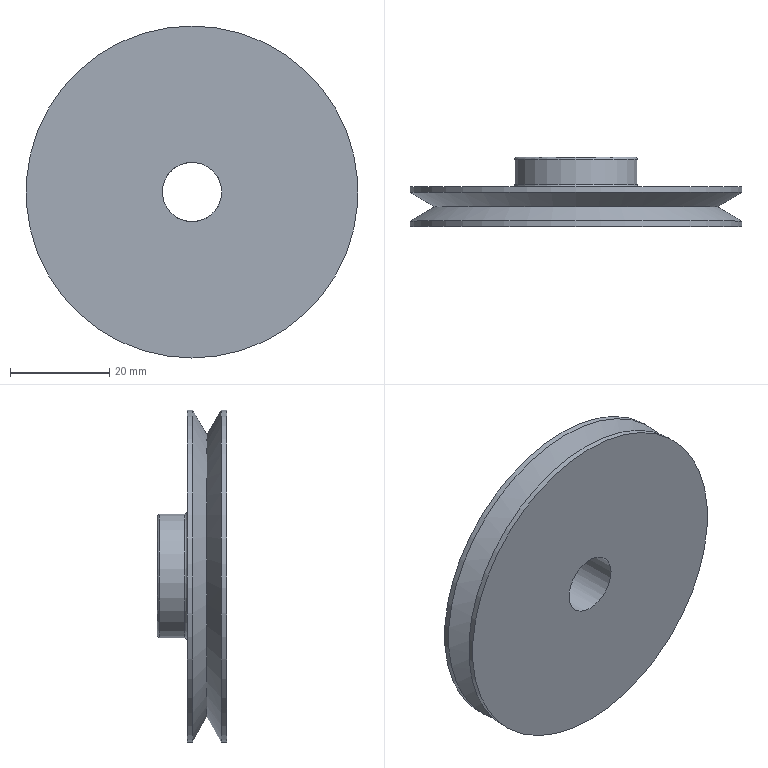Component | NX | PULLEY_2 | 1 solid | 11 faces | box 67 x 14 x 67 mm | volume 26680 mm3 | cylinder 4 | plane 3 | cone 2 | torus 2 | commonest cylinder face diameters 67 x2 25 x1 12 x1
STEP:
#1=CARTESIAN_POINT('',(0.,0.,0.));
#2=DIRECTION('',(0.,0.,1.));
#3=DIRECTION('',(1.,0.,0.));
#4=AXIS2_PLACEMENT_3D('',#1,#2,#3);
#5=CARTESIAN_POINT('',(-218.5,-55.,105.));
#6=VERTEX_POINT('',#5);
#7=CARTESIAN_POINT('',(-212.5,-55.,111.));
#8=VERTEX_POINT('',#7);
#9=CARTESIAN_POINT('',(-218.5,-55.,111.));
#10=DIRECTION('',(0.,-1.,0.));
#11=DIRECTION('',(0.,0.,-1.));
#12=AXIS2_PLACEMENT_3D('',#9,#10,#11);
#13=CIRCLE('',#12,6.);
#14=CARTESIAN_POINT('',(-218.5,-55.,144.5));
#15=DIRECTION('',(0.,-1.,0.));
#16=DIRECTION('',(0.,0.,-1.));
#17=AXIS2_PLACEMENT_3D('',#14,#15,#16);
#18=PLANE('',#17);
#19=CARTESIAN_POINT('',(33.5,0.));
#20=DIRECTION('',(1.,0.));
#21=AXIS2_PLACEMENT_2D('',#19,#20);
#22=CIRCLE('',#21,6.);
#23=(GEOMETRIC_REPRESENTATION_CONTEXT(2)PARAMETRIC_REPRESENTATION_CONTEXT()REPRESENTATION_CONTEXT('',''));
#24=DEFINITIONAL_REPRESENTATION('',(#22),#23);
#25=PCURVE('',#18,#24);
#26=CARTESIAN_POINT('',(-218.5,-96.,111.));
#27=DIRECTION('',(0.,1.,0.));
#28=DIRECTION('',(0.,0.,1.));
#29=AXIS2_PLACEMENT_3D('',#26,#27,#28);
#30=CYLINDRICAL_SURFACE('',#29,6.);
#31=CARTESIAN_POINT('',(3.142,41.));
#32=DIRECTION('',(-1.,0.));
#33=VECTOR('',#32,1.);
#34=LINE('',#31,#33);
#35=(GEOMETRIC_REPRESENTATION_CONTEXT(2)PARAMETRIC_REPRESENTATION_CONTEXT()REPRESENTATION_CONTEXT('',''));
#36=DEFINITIONAL_REPRESENTATION('',(#34),#35);
#37=PCURVE('',#30,#36);
#38=SURFACE_CURVE('',#13,(#25,#37),.PCURVE_S1.);
#39=EDGE_CURVE('',#6,#8,#38,.T.);
#40=ORIENTED_EDGE('',*,*,#39,.F.);
#41=CARTESIAN_POINT('',(-218.5,-55.,111.));
#42=DIRECTION('',(0.,-1.,0.));
#43=DIRECTION('',(0.,0.,-1.));
#44=AXIS2_PLACEMENT_3D('',#41,#42,#43);
#45=CIRCLE('',#44,6.);
#46=CARTESIAN_POINT('',(33.5,0.));
#47=DIRECTION('',(1.,0.));
#48=AXIS2_PLACEMENT_2D('',#46,#47);
#49=CIRCLE('',#48,6.);
#50=(GEOMETRIC_REPRESENTATION_CONTEXT(2)PARAMETRIC_REPRESENTATION_CONTEXT()REPRESENTATION_CONTEXT('',''));
#51=DEFINITIONAL_REPRESENTATION('',(#49),#50);
#52=PCURVE('',#18,#51);
#53=CARTESIAN_POINT('',(9.425,41.));
#54=DIRECTION('',(-1.,0.));
#55=VECTOR('',#54,1.);
#56=LINE('',#53,#55);
#57=(GEOMETRIC_REPRESENTATION_CONTEXT(2)PARAMETRIC_REPRESENTATION_CONTEXT()REPRESENTATION_CONTEXT('',''));
#58=DEFINITIONAL_REPRESENTATION('',(#56),#57);
#59=PCURVE('',#30,#58);
#60=SURFACE_CURVE('',#45,(#52,#59),.PCURVE_S1.);
#61=EDGE_CURVE('',#8,#6,#60,.T.);
#62=ORIENTED_EDGE('',*,*,#61,.F.);
#63=EDGE_LOOP('',(#40,#62));
#64=FACE_BOUND('',#63,.T.);
#65=CARTESIAN_POINT('',(-218.5,-55.,144.5));
#66=VERTEX_POINT('',#65);
#67=CARTESIAN_POINT('',(-218.5,-55.,111.));
#68=DIRECTION('',(0.,1.,0.));
#69=DIRECTION('',(0.,0.,1.));
#70=AXIS2_PLACEMENT_3D('',#67,#68,#69);
#71=CIRCLE('',#70,33.5);
#72=CARTESIAN_POINT('',(0.,0.));
#73=CARTESIAN_POINT('',(0.,58.024));
#74=CARTESIAN_POINT('',(50.25,29.012));
#75=CARTESIAN_POINT('',(100.5,0.));
#76=CARTESIAN_POINT('',(50.25,-29.012));
#77=CARTESIAN_POINT('',(0.,-58.024));
#78=CARTESIAN_POINT('',(0.,0.));
#79=(BOUNDED_CURVE()B_SPLINE_CURVE(2,(#72,#73,#74,#75,#76,#77,#78),.UNSPECIFIED.,.T.,.F.)B_SPLINE_CURVE_WITH_KNOTS((1,2,2,2,2,1),(-2.094,0.,2.094,4.189,6.283,8.378),.UNSPECIFIED.)CURVE()GEOMETRIC_REPRESENTATION_ITEM()RATIONAL_B_SPLINE_CURVE((1.,0.5,1.,0.5,1.,0.5,1.))REPRESENTATION_ITEM(''));
#80=(GEOMETRIC_REPRESENTATION_CONTEXT(2)PARAMETRIC_REPRESENTATION_CONTEXT()REPRESENTATION_CONTEXT('',''));
#81=DEFINITIONAL_REPRESENTATION('',(#79),#80);
#82=PCURVE('',#18,#81);
#83=CARTESIAN_POINT('',(-218.5,-51.,111.));
#84=DIRECTION('',(0.,1.,0.));
#85=DIRECTION('',(0.,0.,1.));
#86=AXIS2_PLACEMENT_3D('',#83,#84,#85);
#87=CYLINDRICAL_SURFACE('',#86,33.5);
#88=CARTESIAN_POINT('',(0.,-4.));
#89=DIRECTION('',(1.,0.));
#90=VECTOR('',#89,1.);
#91=LINE('',#88,#90);
#92=(GEOMETRIC_REPRESENTATION_CONTEXT(2)PARAMETRIC_REPRESENTATION_CONTEXT()REPRESENTATION_CONTEXT('',''));
#93=DEFINITIONAL_REPRESENTATION('',(#91),#92);
#94=PCURVE('',#87,#93);
#95=SURFACE_CURVE('',#71,(#82,#94),.PCURVE_S1.);
#96=EDGE_CURVE('',#66,#66,#95,.T.);
#97=ORIENTED_EDGE('',*,*,#96,.F.);
#98=EDGE_LOOP('',(#97));
#99=FACE_BOUND('',#98,.T.);
#100=ADVANCED_FACE('',(#64,#99),#18,.T.);
#101=ORIENTED_EDGE('',*,*,#96,.T.);
#102=CARTESIAN_POINT('',(-218.5,-53.887,144.5));
#103=VERTEX_POINT('',#102);
#104=CARTESIAN_POINT('',(-218.5,-55.,144.5));
#105=CARTESIAN_POINT('',(-218.5,-53.887,144.5));
#106=B_SPLINE_CURVE_WITH_KNOTS('',1,(#104,#105),.UNSPECIFIED.,.F.,.F.,(2,2),(-4.,-2.887),.PIECEWISE_BEZIER_KNOTS.);
#107=CARTESIAN_POINT('',(6.283,0.));
#108=DIRECTION('',(0.,1.));
#109=VECTOR('',#108,1.);
#110=LINE('',#107,#109);
#111=(GEOMETRIC_REPRESENTATION_CONTEXT(2)PARAMETRIC_REPRESENTATION_CONTEXT()REPRESENTATION_CONTEXT('',''));
#112=DEFINITIONAL_REPRESENTATION('',(#110),#111);
#113=PCURVE('',#87,#112);
#114=CARTESIAN_POINT('',(0.,0.));
#115=DIRECTION('',(0.,1.));
#116=VECTOR('',#115,1.);
#117=LINE('',#114,#116);
#118=(GEOMETRIC_REPRESENTATION_CONTEXT(2)PARAMETRIC_REPRESENTATION_CONTEXT()REPRESENTATION_CONTEXT('',''));
#119=DEFINITIONAL_REPRESENTATION('',(#117),#118);
#120=PCURVE('',#87,#119);
#121=SEAM_CURVE('',#106,(#113,#120),.PCURVE_S1.);
#122=EDGE_CURVE('',#66,#103,#121,.T.);
#123=ORIENTED_EDGE('',*,*,#122,.T.);
#124=CARTESIAN_POINT('',(-218.5,-53.887,111.));
#125=DIRECTION('',(0.,1.,0.));
#126=DIRECTION('',(0.,0.,1.));
#127=AXIS2_PLACEMENT_3D('',#124,#125,#126);
#128=CIRCLE('',#127,33.5);
#129=CARTESIAN_POINT('',(0.,-2.887));
#130=DIRECTION('',(1.,0.));
#131=VECTOR('',#130,1.);
#132=LINE('',#129,#131);
#133=(GEOMETRIC_REPRESENTATION_CONTEXT(2)PARAMETRIC_REPRESENTATION_CONTEXT()REPRESENTATION_CONTEXT('',''));
#134=DEFINITIONAL_REPRESENTATION('',(#132),#133);
#135=PCURVE('',#87,#134);
#136=CARTESIAN_POINT('',(-218.5,-51.,111.));
#137=DIRECTION('',(0.,-1.,0.));
#138=DIRECTION('',(0.,0.,-1.));
#139=AXIS2_PLACEMENT_3D('',#136,#137,#138);
#140=CONICAL_SURFACE('',#139,28.5,1.047);
#141=CARTESIAN_POINT('',(9.425,2.887));
#142=DIRECTION('',(-1.,0.));
#143=VECTOR('',#142,1.);
#144=LINE('',#141,#143);
#145=(GEOMETRIC_REPRESENTATION_CONTEXT(2)PARAMETRIC_REPRESENTATION_CONTEXT()REPRESENTATION_CONTEXT('',''));
#146=DEFINITIONAL_REPRESENTATION('',(#144),#145);
#147=PCURVE('',#140,#146);
#148=SURFACE_CURVE('',#128,(#135,#147),.PCURVE_S1.);
#149=EDGE_CURVE('',#103,#103,#148,.T.);
#150=ORIENTED_EDGE('',*,*,#149,.F.);
#151=ORIENTED_EDGE('',*,*,#122,.F.);
#152=EDGE_LOOP('',(#101,#123,#150,#151));
#153=FACE_BOUND('',#152,.T.);
#154=ADVANCED_FACE('',(#153),#87,.T.);
#155=ORIENTED_EDGE('',*,*,#149,.T.);
#156=CARTESIAN_POINT('',(-218.5,-51.,139.5));
#157=VERTEX_POINT('',#156);
#158=CARTESIAN_POINT('',(-218.5,-51.,139.5));
#159=CARTESIAN_POINT('',(-218.5,-53.887,144.5));
#160=B_SPLINE_CURVE_WITH_KNOTS('',1,(#158,#159),.UNSPECIFIED.,.F.,.F.,(2,2),(0.,5.774),.PIECEWISE_BEZIER_KNOTS.);
#161=CARTESIAN_POINT('',(3.142,0.));
#162=DIRECTION('',(0.,1.));
#163=VECTOR('',#162,1.);
#164=LINE('',#161,#163);
#165=(GEOMETRIC_REPRESENTATION_CONTEXT(2)PARAMETRIC_REPRESENTATION_CONTEXT()REPRESENTATION_CONTEXT('',''));
#166=DEFINITIONAL_REPRESENTATION('',(#164),#165);
#167=PCURVE('',#140,#166);
#168=CARTESIAN_POINT('',(9.425,0.));
#169=DIRECTION('',(0.,1.));
#170=VECTOR('',#169,1.);
#171=LINE('',#168,#170);
#172=(GEOMETRIC_REPRESENTATION_CONTEXT(2)PARAMETRIC_REPRESENTATION_CONTEXT()REPRESENTATION_CONTEXT('',''));
#173=DEFINITIONAL_REPRESENTATION('',(#171),#172);
#174=PCURVE('',#140,#173);
#175=SEAM_CURVE('',#160,(#167,#174),.PCURVE_S1.);
#176=EDGE_CURVE('',#157,#103,#175,.T.);
#177=ORIENTED_EDGE('',*,*,#176,.F.);
#178=CARTESIAN_POINT('',(-218.5,-51.,111.));
#179=DIRECTION('',(0.,1.,0.));
#180=DIRECTION('',(0.,0.,1.));
#181=AXIS2_PLACEMENT_3D('',#178,#179,#180);
#182=CIRCLE('',#181,28.5);
#183=CARTESIAN_POINT('',(9.425,0.));
#184=DIRECTION('',(-1.,0.));
#185=VECTOR('',#184,1.);
#186=LINE('',#183,#185);
#187=(GEOMETRIC_REPRESENTATION_CONTEXT(2)PARAMETRIC_REPRESENTATION_CONTEXT()REPRESENTATION_CONTEXT('',''));
#188=DEFINITIONAL_REPRESENTATION('',(#186),#187);
#189=PCURVE('',#140,#188);
#190=CARTESIAN_POINT('',(-218.5,-48.113,111.));
#191=DIRECTION('',(0.,1.,0.));
#192=DIRECTION('',(0.,0.,1.));
#193=AXIS2_PLACEMENT_3D('',#190,#191,#192);
#194=CONICAL_SURFACE('',#193,33.5,1.047);
#195=CARTESIAN_POINT('',(0.,-2.887));
#196=DIRECTION('',(1.,0.));
#197=VECTOR('',#196,1.);
#198=LINE('',#195,#197);
#199=(GEOMETRIC_REPRESENTATION_CONTEXT(2)PARAMETRIC_REPRESENTATION_CONTEXT()REPRESENTATION_CONTEXT('',''));
#200=DEFINITIONAL_REPRESENTATION('',(#198),#199);
#201=PCURVE('',#194,#200);
#202=SURFACE_CURVE('',#182,(#189,#201),.PCURVE_S1.);
#203=EDGE_CURVE('',#157,#157,#202,.T.);
#204=ORIENTED_EDGE('',*,*,#203,.F.);
#205=ORIENTED_EDGE('',*,*,#176,.T.);
#206=EDGE_LOOP('',(#155,#177,#204,#205));
#207=FACE_BOUND('',#206,.T.);
#208=ADVANCED_FACE('',(#207),#140,.T.);
#209=ORIENTED_EDGE('',*,*,#203,.T.);
#210=CARTESIAN_POINT('',(-218.5,-48.113,144.5));
#211=VERTEX_POINT('',#210);
#212=CARTESIAN_POINT('',(-218.5,-51.,139.5));
#213=CARTESIAN_POINT('',(-218.5,-48.113,144.5));
#214=B_SPLINE_CURVE_WITH_KNOTS('',1,(#212,#213),.UNSPECIFIED.,.F.,.F.,(2,2),(-5.774,0.),.PIECEWISE_BEZIER_KNOTS.);
#215=CARTESIAN_POINT('',(6.283,0.));
#216=DIRECTION('',(0.,1.));
#217=VECTOR('',#216,1.);
#218=LINE('',#215,#217);
#219=(GEOMETRIC_REPRESENTATION_CONTEXT(2)PARAMETRIC_REPRESENTATION_CONTEXT()REPRESENTATION_CONTEXT('',''));
#220=DEFINITIONAL_REPRESENTATION('',(#218),#219);
#221=PCURVE('',#194,#220);
#222=CARTESIAN_POINT('',(0.,0.));
#223=DIRECTION('',(0.,1.));
#224=VECTOR('',#223,1.);
#225=LINE('',#222,#224);
#226=(GEOMETRIC_REPRESENTATION_CONTEXT(2)PARAMETRIC_REPRESENTATION_CONTEXT()REPRESENTATION_CONTEXT('',''));
#227=DEFINITIONAL_REPRESENTATION('',(#225),#226);
#228=PCURVE('',#194,#227);
#229=SEAM_CURVE('',#214,(#221,#228),.PCURVE_S1.);
#230=EDGE_CURVE('',#157,#211,#229,.T.);
#231=ORIENTED_EDGE('',*,*,#230,.T.);
#232=CARTESIAN_POINT('',(-218.5,-48.113,111.));
#233=DIRECTION('',(0.,1.,0.));
#234=DIRECTION('',(0.,0.,1.));
#235=AXIS2_PLACEMENT_3D('',#232,#233,#234);
#236=CIRCLE('',#235,33.5);
#237=CARTESIAN_POINT('',(0.,0.));
#238=DIRECTION('',(1.,0.));
#239=VECTOR('',#238,1.);
#240=LINE('',#237,#239);
#241=(GEOMETRIC_REPRESENTATION_CONTEXT(2)PARAMETRIC_REPRESENTATION_CONTEXT()REPRESENTATION_CONTEXT('',''));
#242=DEFINITIONAL_REPRESENTATION('',(#240),#241);
#243=PCURVE('',#194,#242);
#244=CARTESIAN_POINT('',(-218.5,-51.,111.));
#245=DIRECTION('',(0.,1.,0.));
#246=DIRECTION('',(0.,0.,1.));
#247=AXIS2_PLACEMENT_3D('',#244,#245,#246);
#248=CYLINDRICAL_SURFACE('',#247,33.5);
#249=CARTESIAN_POINT('',(0.,2.887));
#250=DIRECTION('',(1.,0.));
#251=VECTOR('',#250,1.);
#252=LINE('',#249,#251);
#253=(GEOMETRIC_REPRESENTATION_CONTEXT(2)PARAMETRIC_REPRESENTATION_CONTEXT()REPRESENTATION_CONTEXT('',''));
#254=DEFINITIONAL_REPRESENTATION('',(#252),#253);
#255=PCURVE('',#248,#254);
#256=SURFACE_CURVE('',#236,(#243,#255),.PCURVE_S1.);
#257=EDGE_CURVE('',#211,#211,#256,.T.);
#258=ORIENTED_EDGE('',*,*,#257,.F.);
#259=ORIENTED_EDGE('',*,*,#230,.F.);
#260=EDGE_LOOP('',(#209,#231,#258,#259));
#261=FACE_BOUND('',#260,.T.);
#262=ADVANCED_FACE('',(#261),#194,.T.);
#263=ORIENTED_EDGE('',*,*,#257,.T.);
#264=CARTESIAN_POINT('',(-218.5,-47.,144.5));
#265=VERTEX_POINT('',#264);
#266=CARTESIAN_POINT('',(-218.5,-48.113,144.5));
#267=CARTESIAN_POINT('',(-218.5,-47.,144.5));
#268=B_SPLINE_CURVE_WITH_KNOTS('',1,(#266,#267),.UNSPECIFIED.,.F.,.F.,(2,2),(2.887,4.),.PIECEWISE_BEZIER_KNOTS.);
#269=CARTESIAN_POINT('',(6.283,0.));
#270=DIRECTION('',(0.,1.));
#271=VECTOR('',#270,1.);
#272=LINE('',#269,#271);
#273=(GEOMETRIC_REPRESENTATION_CONTEXT(2)PARAMETRIC_REPRESENTATION_CONTEXT()REPRESENTATION_CONTEXT('',''));
#274=DEFINITIONAL_REPRESENTATION('',(#272),#273);
#275=PCURVE('',#248,#274);
#276=CARTESIAN_POINT('',(0.,0.));
#277=DIRECTION('',(0.,1.));
#278=VECTOR('',#277,1.);
#279=LINE('',#276,#278);
#280=(GEOMETRIC_REPRESENTATION_CONTEXT(2)PARAMETRIC_REPRESENTATION_CONTEXT()REPRESENTATION_CONTEXT('',''));
#281=DEFINITIONAL_REPRESENTATION('',(#279),#280);
#282=PCURVE('',#248,#281);
#283=SEAM_CURVE('',#268,(#275,#282),.PCURVE_S1.);
#284=EDGE_CURVE('',#211,#265,#283,.T.);
#285=ORIENTED_EDGE('',*,*,#284,.T.);
#286=CARTESIAN_POINT('',(-218.5,-47.,111.));
#287=DIRECTION('',(0.,1.,0.));
#288=DIRECTION('',(0.,0.,1.));
#289=AXIS2_PLACEMENT_3D('',#286,#287,#288);
#290=CIRCLE('',#289,33.5);
#291=CARTESIAN_POINT('',(0.,4.));
#292=DIRECTION('',(1.,0.));
#293=VECTOR('',#292,1.);
#294=LINE('',#291,#293);
#295=(GEOMETRIC_REPRESENTATION_CONTEXT(2)PARAMETRIC_REPRESENTATION_CONTEXT()REPRESENTATION_CONTEXT('',''));
#296=DEFINITIONAL_REPRESENTATION('',(#294),#295);
#297=PCURVE('',#248,#296);
#298=CARTESIAN_POINT('',(-218.5,-47.,111.));
#299=DIRECTION('',(0.,1.,0.));
#300=DIRECTION('',(0.,0.,1.));
#301=AXIS2_PLACEMENT_3D('',#298,#299,#300);
#302=PLANE('',#301);
#303=CARTESIAN_POINT('',(0.,0.));
#304=DIRECTION('',(1.,0.));
#305=AXIS2_PLACEMENT_2D('',#303,#304);
#306=CIRCLE('',#305,33.5);
#307=(GEOMETRIC_REPRESENTATION_CONTEXT(2)PARAMETRIC_REPRESENTATION_CONTEXT()REPRESENTATION_CONTEXT('',''));
#308=DEFINITIONAL_REPRESENTATION('',(#306),#307);
#309=PCURVE('',#302,#308);
#310=SURFACE_CURVE('',#290,(#297,#309),.PCURVE_S1.);
#311=EDGE_CURVE('',#265,#265,#310,.T.);
#312=ORIENTED_EDGE('',*,*,#311,.F.);
#313=ORIENTED_EDGE('',*,*,#284,.F.);
#314=EDGE_LOOP('',(#263,#285,#312,#313));
#315=FACE_BOUND('',#314,.T.);
#316=ADVANCED_FACE('',(#315),#248,.T.);
#317=CARTESIAN_POINT('',(-218.5,-47.,124.));
#318=VERTEX_POINT('',#317);
#319=CARTESIAN_POINT('',(-218.5,-47.,111.));
#320=DIRECTION('',(0.,-1.,0.));
#321=DIRECTION('',(0.,0.,1.));
#322=AXIS2_PLACEMENT_3D('',#319,#320,#321);
#323=CIRCLE('',#322,13.);
#324=CARTESIAN_POINT('',(13.,0.));
#325=CARTESIAN_POINT('',(13.,-22.517));
#326=CARTESIAN_POINT('',(-6.5,-11.258));
#327=CARTESIAN_POINT('',(-26.,-0.));
#328=CARTESIAN_POINT('',(-6.5,11.258));
#329=CARTESIAN_POINT('',(13.,22.517));
#330=CARTESIAN_POINT('',(13.,0.));
#331=(BOUNDED_CURVE()B_SPLINE_CURVE(2,(#324,#325,#326,#327,#328,#329,#330),.UNSPECIFIED.,.T.,.F.)B_SPLINE_CURVE_WITH_KNOTS((1,2,2,2,2,1),(-2.094,0.,2.094,4.189,6.283,8.378),.UNSPECIFIED.)CURVE()GEOMETRIC_REPRESENTATION_ITEM()RATIONAL_B_SPLINE_CURVE((1.,0.5,1.,0.5,1.,0.5,1.))REPRESENTATION_ITEM(''));
#332=(GEOMETRIC_REPRESENTATION_CONTEXT(2)PARAMETRIC_REPRESENTATION_CONTEXT()REPRESENTATION_CONTEXT('',''));
#333=DEFINITIONAL_REPRESENTATION('',(#331),#332);
#334=PCURVE('',#302,#333);
#335=CARTESIAN_POINT('',(-218.5,-46.5,111.));
#336=DIRECTION('',(0.,1.,0.));
#337=DIRECTION('',(0.,0.,1.));
#338=AXIS2_PLACEMENT_3D('',#335,#336,#337);
#339=TOROIDAL_SURFACE('',#338,13.,0.5);
#340=CARTESIAN_POINT('',(6.283,4.712));
#341=DIRECTION('',(-1.,0.));
#342=VECTOR('',#341,1.);
#343=LINE('',#340,#342);
#344=(GEOMETRIC_REPRESENTATION_CONTEXT(2)PARAMETRIC_REPRESENTATION_CONTEXT()REPRESENTATION_CONTEXT('',''));
#345=DEFINITIONAL_REPRESENTATION('',(#343),#344);
#346=PCURVE('',#339,#345);
#347=SURFACE_CURVE('',#323,(#334,#346),.PCURVE_S1.);
#348=EDGE_CURVE('',#318,#318,#347,.T.);
#349=ORIENTED_EDGE('',*,*,#348,.T.);
#350=EDGE_LOOP('',(#349));
#351=FACE_BOUND('',#350,.T.);
#352=ORIENTED_EDGE('',*,*,#311,.T.);
#353=EDGE_LOOP('',(#352));
#354=FACE_BOUND('',#353,.T.);
#355=ADVANCED_FACE('',(#351,#354),#302,.T.);
#356=CARTESIAN_POINT('',(-212.5,-41.,111.));
#357=VERTEX_POINT('',#356);
#358=CARTESIAN_POINT('',(-218.5,-41.,111.));
#359=DIRECTION('',(0.,1.,0.));
#360=DIRECTION('',(1.,0.,0.));
#361=AXIS2_PLACEMENT_3D('',#358,#359,#360);
#362=CIRCLE('',#361,6.);
#363=CARTESIAN_POINT('',(-218.5,-41.,111.));
#364=DIRECTION('',(0.,1.,0.));
#365=DIRECTION('',(0.,0.,1.));
#366=AXIS2_PLACEMENT_3D('',#363,#364,#365);
#367=PLANE('',#366);
#368=CARTESIAN_POINT('',(0.,0.));
#369=DIRECTION('',(0.,1.));
#370=AXIS2_PLACEMENT_2D('',#368,#369);
#371=CIRCLE('',#370,6.);
#372=(GEOMETRIC_REPRESENTATION_CONTEXT(2)PARAMETRIC_REPRESENTATION_CONTEXT()REPRESENTATION_CONTEXT('',''));
#373=DEFINITIONAL_REPRESENTATION('',(#371),#372);
#374=PCURVE('',#367,#373);
#375=CARTESIAN_POINT('',(1.571,55.));
#376=DIRECTION('',(1.,0.));
#377=VECTOR('',#376,1.);
#378=LINE('',#375,#377);
#379=(GEOMETRIC_REPRESENTATION_CONTEXT(2)PARAMETRIC_REPRESENTATION_CONTEXT()REPRESENTATION_CONTEXT('',''));
#380=DEFINITIONAL_REPRESENTATION('',(#378),#379);
#381=PCURVE('',#30,#380);
#382=SURFACE_CURVE('',#362,(#374,#381),.PCURVE_S1.);
#383=EDGE_CURVE('',#357,#357,#382,.T.);
#384=ORIENTED_EDGE('',*,*,#383,.F.);
#385=EDGE_LOOP('',(#384));
#386=FACE_BOUND('',#385,.T.);
#387=CARTESIAN_POINT('',(-218.5,-41.,123.));
#388=VERTEX_POINT('',#387);
#389=CARTESIAN_POINT('',(-218.5,-41.,111.));
#390=DIRECTION('',(0.,1.,0.));
#391=DIRECTION('',(0.,0.,1.));
#392=AXIS2_PLACEMENT_3D('',#389,#390,#391);
#393=CIRCLE('',#392,12.);
#394=CARTESIAN_POINT('',(0.,0.));
#395=DIRECTION('',(1.,0.));
#396=AXIS2_PLACEMENT_2D('',#394,#395);
#397=CIRCLE('',#396,12.);
#398=(GEOMETRIC_REPRESENTATION_CONTEXT(2)PARAMETRIC_REPRESENTATION_CONTEXT()REPRESENTATION_CONTEXT('',''));
#399=DEFINITIONAL_REPRESENTATION('',(#397),#398);
#400=PCURVE('',#367,#399);
#401=CARTESIAN_POINT('',(-218.5,-41.5,111.));
#402=DIRECTION('',(0.,1.,0.));
#403=DIRECTION('',(0.,0.,1.));
#404=AXIS2_PLACEMENT_3D('',#401,#402,#403);
#405=TOROIDAL_SURFACE('',#404,12.,0.5);
#406=CARTESIAN_POINT('',(0.,7.854));
#407=DIRECTION('',(1.,0.));
#408=VECTOR('',#407,1.);
#409=LINE('',#406,#408);
#410=(GEOMETRIC_REPRESENTATION_CONTEXT(2)PARAMETRIC_REPRESENTATION_CONTEXT()REPRESENTATION_CONTEXT('',''));
#411=DEFINITIONAL_REPRESENTATION('',(#409),#410);
#412=PCURVE('',#405,#411);
#413=SURFACE_CURVE('',#393,(#400,#412),.PCURVE_S1.);
#414=EDGE_CURVE('',#388,#388,#413,.T.);
#415=ORIENTED_EDGE('',*,*,#414,.T.);
#416=EDGE_LOOP('',(#415));
#417=FACE_BOUND('',#416,.T.);
#418=ADVANCED_FACE('',(#386,#417),#367,.T.);
#419=CARTESIAN_POINT('',(-218.5,-46.5,123.5));
#420=VERTEX_POINT('',#419);
#421=CARTESIAN_POINT('',(-218.5,-46.5,111.));
#422=DIRECTION('',(0.,1.,0.));
#423=DIRECTION('',(0.,0.,1.));
#424=AXIS2_PLACEMENT_3D('',#421,#422,#423);
#425=CIRCLE('',#424,12.5);
#426=CARTESIAN_POINT('',(-218.5,-47.,111.));
#427=DIRECTION('',(0.,1.,0.));
#428=DIRECTION('',(0.,0.,1.));
#429=AXIS2_PLACEMENT_3D('',#426,#427,#428);
#430=CYLINDRICAL_SURFACE('',#429,12.5);
#431=CARTESIAN_POINT('',(0.,0.5));
#432=DIRECTION('',(1.,0.));
#433=VECTOR('',#432,1.);
#434=LINE('',#431,#433);
#435=(GEOMETRIC_REPRESENTATION_CONTEXT(2)PARAMETRIC_REPRESENTATION_CONTEXT()REPRESENTATION_CONTEXT('',''));
#436=DEFINITIONAL_REPRESENTATION('',(#434),#435);
#437=PCURVE('',#430,#436);
#438=CARTESIAN_POINT('',(0.,3.142));
#439=DIRECTION('',(1.,0.));
#440=VECTOR('',#439,1.);
#441=LINE('',#438,#440);
#442=(GEOMETRIC_REPRESENTATION_CONTEXT(2)PARAMETRIC_REPRESENTATION_CONTEXT()REPRESENTATION_CONTEXT('',''));
#443=DEFINITIONAL_REPRESENTATION('',(#441),#442);
#444=PCURVE('',#339,#443);
#445=SURFACE_CURVE('',#425,(#437,#444),.PCURVE_S1.);
#446=EDGE_CURVE('',#420,#420,#445,.T.);
#447=ORIENTED_EDGE('',*,*,#446,.T.);
#448=CARTESIAN_POINT('',(-218.5,-41.5,123.5));
#449=VERTEX_POINT('',#448);
#450=CARTESIAN_POINT('',(-218.5,-46.5,123.5));
#451=CARTESIAN_POINT('',(-218.5,-41.5,123.5));
#452=B_SPLINE_CURVE_WITH_KNOTS('',1,(#450,#451),.UNSPECIFIED.,.F.,.F.,(2,2),(0.5,5.5),.PIECEWISE_BEZIER_KNOTS.);
#453=CARTESIAN_POINT('',(6.283,0.));
#454=DIRECTION('',(0.,1.));
#455=VECTOR('',#454,1.);
#456=LINE('',#453,#455);
#457=(GEOMETRIC_REPRESENTATION_CONTEXT(2)PARAMETRIC_REPRESENTATION_CONTEXT()REPRESENTATION_CONTEXT('',''));
#458=DEFINITIONAL_REPRESENTATION('',(#456),#457);
#459=PCURVE('',#430,#458);
#460=CARTESIAN_POINT('',(0.,0.));
#461=DIRECTION('',(0.,1.));
#462=VECTOR('',#461,1.);
#463=LINE('',#460,#462);
#464=(GEOMETRIC_REPRESENTATION_CONTEXT(2)PARAMETRIC_REPRESENTATION_CONTEXT()REPRESENTATION_CONTEXT('',''));
#465=DEFINITIONAL_REPRESENTATION('',(#463),#464);
#466=PCURVE('',#430,#465);
#467=SEAM_CURVE('',#452,(#459,#466),.PCURVE_S1.);
#468=EDGE_CURVE('',#420,#449,#467,.T.);
#469=ORIENTED_EDGE('',*,*,#468,.T.);
#470=CARTESIAN_POINT('',(-218.5,-41.5,111.));
#471=DIRECTION('',(0.,-1.,0.));
#472=DIRECTION('',(0.,0.,1.));
#473=AXIS2_PLACEMENT_3D('',#470,#471,#472);
#474=CIRCLE('',#473,12.5);
#475=CARTESIAN_POINT('',(6.283,5.5));
#476=DIRECTION('',(-1.,0.));
#477=VECTOR('',#476,1.);
#478=LINE('',#475,#477);
#479=(GEOMETRIC_REPRESENTATION_CONTEXT(2)PARAMETRIC_REPRESENTATION_CONTEXT()REPRESENTATION_CONTEXT('',''));
#480=DEFINITIONAL_REPRESENTATION('',(#478),#479);
#481=PCURVE('',#430,#480);
#482=CARTESIAN_POINT('',(6.283,6.283));
#483=DIRECTION('',(-1.,0.));
#484=VECTOR('',#483,1.);
#485=LINE('',#482,#484);
#486=(GEOMETRIC_REPRESENTATION_CONTEXT(2)PARAMETRIC_REPRESENTATION_CONTEXT()REPRESENTATION_CONTEXT('',''));
#487=DEFINITIONAL_REPRESENTATION('',(#485),#486);
#488=PCURVE('',#405,#487);
#489=SURFACE_CURVE('',#474,(#481,#488),.PCURVE_S1.);
#490=EDGE_CURVE('',#449,#449,#489,.T.);
#491=ORIENTED_EDGE('',*,*,#490,.T.);
#492=ORIENTED_EDGE('',*,*,#468,.F.);
#493=EDGE_LOOP('',(#447,#469,#491,#492));
#494=FACE_BOUND('',#493,.T.);
#495=ADVANCED_FACE('',(#494),#430,.T.);
#496=ORIENTED_EDGE('',*,*,#348,.T.);
#497=CARTESIAN_POINT('',(-218.5,-46.5,123.5));
#498=CARTESIAN_POINT('',(-218.5,-46.634,123.5));
#499=CARTESIAN_POINT('',(-218.5,-46.764,123.543));
#500=CARTESIAN_POINT('',(-218.5,-46.876,123.624));
#501=CARTESIAN_POINT('',(-218.5,-46.957,123.736));
#502=CARTESIAN_POINT('',(-218.5,-47.,123.866));
#503=CARTESIAN_POINT('',(-218.5,-47.,124.));
#504=(BOUNDED_CURVE()B_SPLINE_CURVE(6,(#497,#498,#499,#500,#501,#502,#503),.UNSPECIFIED.,.F.,.F.)B_SPLINE_CURVE_WITH_KNOTS((7,7),(3.142,4.712),.PIECEWISE_BEZIER_KNOTS.)CURVE()GEOMETRIC_REPRESENTATION_ITEM()RATIONAL_B_SPLINE_CURVE((1.031,1.01,0.9979,0.994,0.9979,1.01,1.031))REPRESENTATION_ITEM(''));
#505=CARTESIAN_POINT('',(0.,0.));
#506=DIRECTION('',(0.,1.));
#507=VECTOR('',#506,1.);
#508=LINE('',#505,#507);
#509=(GEOMETRIC_REPRESENTATION_CONTEXT(2)PARAMETRIC_REPRESENTATION_CONTEXT()REPRESENTATION_CONTEXT('',''));
#510=DEFINITIONAL_REPRESENTATION('',(#508),#509);
#511=PCURVE('',#339,#510);
#512=CARTESIAN_POINT('',(6.283,0.));
#513=DIRECTION('',(0.,1.));
#514=VECTOR('',#513,1.);
#515=LINE('',#512,#514);
#516=(GEOMETRIC_REPRESENTATION_CONTEXT(2)PARAMETRIC_REPRESENTATION_CONTEXT()REPRESENTATION_CONTEXT('',''));
#517=DEFINITIONAL_REPRESENTATION('',(#515),#516);
#518=PCURVE('',#339,#517);
#519=SEAM_CURVE('',#504,(#511,#518),.PCURVE_S1.);
#520=EDGE_CURVE('',#420,#318,#519,.T.);
#521=ORIENTED_EDGE('',*,*,#520,.F.);
#522=ORIENTED_EDGE('',*,*,#446,.T.);
#523=ORIENTED_EDGE('',*,*,#520,.T.);
#524=EDGE_LOOP('',(#496,#521,#522,#523));
#525=FACE_BOUND('',#524,.F.);
#526=ADVANCED_FACE('',(#525),#339,.F.);
#527=ORIENTED_EDGE('',*,*,#490,.F.);
#528=CARTESIAN_POINT('',(-218.5,-41.5,123.5));
#529=CARTESIAN_POINT('',(-218.5,-41.366,123.5));
#530=CARTESIAN_POINT('',(-218.5,-41.236,123.457));
#531=CARTESIAN_POINT('',(-218.5,-41.124,123.376));
#532=CARTESIAN_POINT('',(-218.5,-41.043,123.264));
#533=CARTESIAN_POINT('',(-218.5,-41.,123.134));
#534=CARTESIAN_POINT('',(-218.5,-41.,123.));
#535=(BOUNDED_CURVE()B_SPLINE_CURVE(6,(#528,#529,#530,#531,#532,#533,#534),.UNSPECIFIED.,.F.,.F.)B_SPLINE_CURVE_WITH_KNOTS((7,7),(0.,1.571),.PIECEWISE_BEZIER_KNOTS.)CURVE()GEOMETRIC_REPRESENTATION_ITEM()RATIONAL_B_SPLINE_CURVE((1.031,1.01,0.9979,0.994,0.9979,1.01,1.031))REPRESENTATION_ITEM(''));
#536=CARTESIAN_POINT('',(6.283,6.283));
#537=DIRECTION('',(0.,1.));
#538=VECTOR('',#537,1.);
#539=LINE('',#536,#538);
#540=(GEOMETRIC_REPRESENTATION_CONTEXT(2)PARAMETRIC_REPRESENTATION_CONTEXT()REPRESENTATION_CONTEXT('',''));
#541=DEFINITIONAL_REPRESENTATION('',(#539),#540);
#542=PCURVE('',#405,#541);
#543=CARTESIAN_POINT('',(0.,6.283));
#544=DIRECTION('',(0.,1.));
#545=VECTOR('',#544,1.);
#546=LINE('',#543,#545);
#547=(GEOMETRIC_REPRESENTATION_CONTEXT(2)PARAMETRIC_REPRESENTATION_CONTEXT()REPRESENTATION_CONTEXT('',''));
#548=DEFINITIONAL_REPRESENTATION('',(#546),#547);
#549=PCURVE('',#405,#548);
#550=SEAM_CURVE('',#535,(#542,#549),.PCURVE_S1.);
#551=EDGE_CURVE('',#449,#388,#550,.T.);
#552=ORIENTED_EDGE('',*,*,#551,.T.);
#553=ORIENTED_EDGE('',*,*,#414,.F.);
#554=ORIENTED_EDGE('',*,*,#551,.F.);
#555=EDGE_LOOP('',(#527,#552,#553,#554));
#556=FACE_BOUND('',#555,.T.);
#557=ADVANCED_FACE('',(#556),#405,.T.);
#558=ORIENTED_EDGE('',*,*,#61,.F.);
#559=CARTESIAN_POINT('',(-212.5,-55.,111.));
#560=CARTESIAN_POINT('',(-212.5,-41.,111.));
#561=B_SPLINE_CURVE_WITH_KNOTS('',1,(#559,#560),.UNSPECIFIED.,.F.,.F.,(2,2),(41.,55.),.PIECEWISE_BEZIER_KNOTS.);
#562=CARTESIAN_POINT('',(7.854,0.));
#563=DIRECTION('',(0.,1.));
#564=VECTOR('',#563,1.);
#565=LINE('',#562,#564);
#566=(GEOMETRIC_REPRESENTATION_CONTEXT(2)PARAMETRIC_REPRESENTATION_CONTEXT()REPRESENTATION_CONTEXT('',''));
#567=DEFINITIONAL_REPRESENTATION('',(#565),#566);
#568=PCURVE('',#30,#567);
#569=CARTESIAN_POINT('',(1.571,0.));
#570=DIRECTION('',(0.,1.));
#571=VECTOR('',#570,1.);
#572=LINE('',#569,#571);
#573=(GEOMETRIC_REPRESENTATION_CONTEXT(2)PARAMETRIC_REPRESENTATION_CONTEXT()REPRESENTATION_CONTEXT('',''));
#574=DEFINITIONAL_REPRESENTATION('',(#572),#573);
#575=PCURVE('',#30,#574);
#576=SEAM_CURVE('',#561,(#568,#575),.PCURVE_S1.);
#577=EDGE_CURVE('',#8,#357,#576,.T.);
#578=ORIENTED_EDGE('',*,*,#577,.T.);
#579=ORIENTED_EDGE('',*,*,#383,.F.);
#580=ORIENTED_EDGE('',*,*,#577,.F.);
#581=ORIENTED_EDGE('',*,*,#39,.F.);
#582=EDGE_LOOP('',(#558,#578,#579,#580,#581));
#583=FACE_BOUND('',#582,.F.);
#584=ADVANCED_FACE('',(#583),#30,.F.);
#585=CLOSED_SHELL('',(#100,#154,#208,#262,#316,#355,#418,#495,#526,#557,#584));
#586=MANIFOLD_SOLID_BREP('',#585);
#587=(LENGTH_UNIT()NAMED_UNIT(*)SI_UNIT(.MILLI.,.METRE.));
#588=UNCERTAINTY_MEASURE_WITH_UNIT(LENGTH_MEASURE(0.00001),#587,'','');
#589=(NAMED_UNIT(*)PLANE_ANGLE_UNIT()SI_UNIT($,.RADIAN.));
#590=(NAMED_UNIT(*)SI_UNIT($,.STERADIAN.)SOLID_ANGLE_UNIT());
#591=(GEOMETRIC_REPRESENTATION_CONTEXT(3)GLOBAL_UNCERTAINTY_ASSIGNED_CONTEXT((#588))GLOBAL_UNIT_ASSIGNED_CONTEXT((#587,#589,#590))REPRESENTATION_CONTEXT('',''));
#592=ADVANCED_BREP_SHAPE_REPRESENTATION('',(#4,#586),#591);